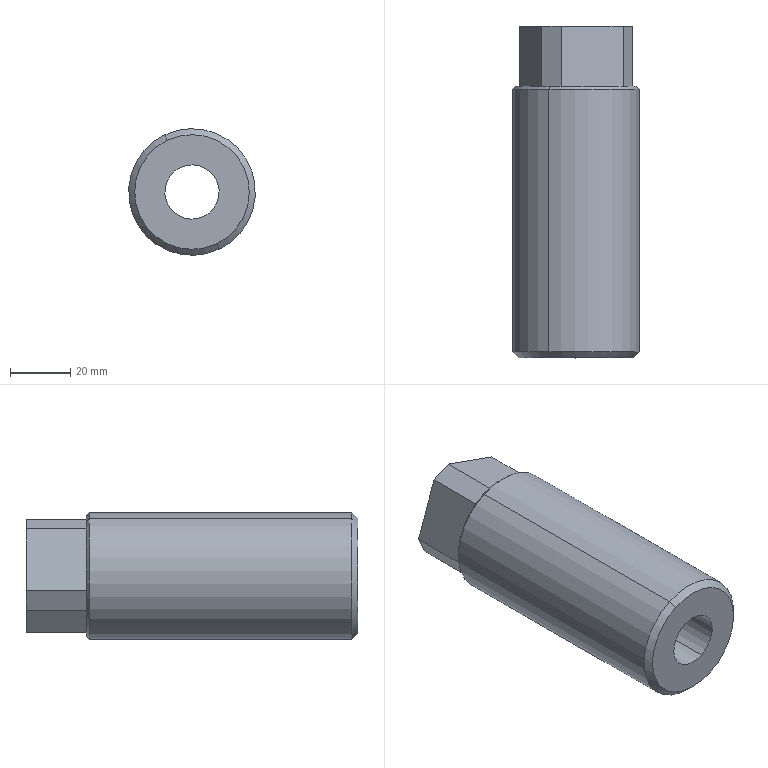Component | SolidWorks | YC1-250-02-28MotorSeatAssembly-1_YC1-200-02-29AdjustmentScrew-1 | 1 solid | 19 faces | box 42 x 110 x 42 mm | volume 115805 mm3 | plane 11 | cylinder 4 | cone 4 | commonest cylinder face diameters 42 x2 18 x2 | material Plain Carbon Steel
STEP:
#1=CARTESIAN_POINT('',(15.592,146.811,-50.827));
#2=VERTEX_POINT('',#1);
#3=CARTESIAN_POINT('',(16.298,146.811,-52.322));
#4=VERTEX_POINT('',#3);
#5=CARTESIAN_POINT('',(15.945,146.811,-51.575));
#6=DIRECTION('',(0.,-1.,0.));
#7=DIRECTION('',(-0.4273,0.,0.9041));
#8=AXIS2_PLACEMENT_3D('',#5,#6,#7);
#9=CIRCLE('',#8,0.8268);
#10=EDGE_CURVE('',#2,#4,#9,.T.);
#11=ORIENTED_EDGE('',*,*,#10,.T.);
#12=CARTESIAN_POINT('',(16.298,143.386,-52.322));
#13=VERTEX_POINT('',#12);
#14=CARTESIAN_POINT('',(16.298,147.638,-52.322));
#15=DIRECTION('',(0.,-1.,0.));
#16=VECTOR('',#15,39.37);
#17=LINE('',#14,#16);
#18=EDGE_CURVE('',#4,#13,#17,.T.);
#19=ORIENTED_EDGE('',*,*,#18,.T.);
#20=CARTESIAN_POINT('',(15.592,143.386,-50.827));
#21=VERTEX_POINT('',#20);
#22=CARTESIAN_POINT('',(15.945,143.386,-51.575));
#23=DIRECTION('',(0.,1.,0.));
#24=DIRECTION('',(-0.4273,0.,0.9041));
#25=AXIS2_PLACEMENT_3D('',#22,#23,#24);
#26=CIRCLE('',#25,0.8268);
#27=EDGE_CURVE('',#13,#21,#26,.T.);
#28=ORIENTED_EDGE('',*,*,#27,.T.);
#29=CARTESIAN_POINT('',(15.592,147.638,-50.827));
#30=DIRECTION('',(0.,-1.,0.));
#31=VECTOR('',#30,39.37);
#32=LINE('',#29,#31);
#33=EDGE_CURVE('',#2,#21,#32,.T.);
#34=ORIENTED_EDGE('',*,*,#33,.F.);
#35=EDGE_LOOP('',(#11,#19,#28,#34));
#36=FACE_OUTER_BOUND('',#35,.T.);
#37=CARTESIAN_POINT('',(15.945,147.638,-51.575));
#38=DIRECTION('',(0.,-1.,0.));
#39=DIRECTION('',(-0.4273,0.,0.9041));
#40=AXIS2_PLACEMENT_3D('',#37,#38,#39);
#41=CYLINDRICAL_SURFACE('',#40,0.8268);
#42=ADVANCED_FACE('',(#36),#41,.T.);
#43=CARTESIAN_POINT('',(16.264,143.307,-52.251));
#44=VERTEX_POINT('',#43);
#45=CARTESIAN_POINT('',(15.625,143.307,-50.898));
#46=VERTEX_POINT('',#45);
#47=CARTESIAN_POINT('',(15.945,143.307,-51.575));
#48=DIRECTION('',(0.,1.,0.));
#49=DIRECTION('',(0.4273,0.,-0.9041));
#50=AXIS2_PLACEMENT_3D('',#47,#48,#49);
#51=CIRCLE('',#50,0.748);
#52=EDGE_CURVE('',#44,#46,#51,.T.);
#53=ORIENTED_EDGE('',*,*,#52,.T.);
#54=CARTESIAN_POINT('',(15.592,143.386,-50.827));
#55=DIRECTION('',(-0.3021,0.7071,0.6393));
#56=VECTOR('',#55,39.37);
#57=LINE('',#54,#56);
#58=EDGE_CURVE('',#46,#21,#57,.T.);
#59=ORIENTED_EDGE('',*,*,#58,.T.);
#60=ORIENTED_EDGE('',*,*,#27,.F.);
#61=CARTESIAN_POINT('',(16.298,143.386,-52.322));
#62=DIRECTION('',(0.3021,0.7071,-0.6393));
#63=VECTOR('',#62,39.37);
#64=LINE('',#61,#63);
#65=EDGE_CURVE('',#44,#13,#64,.T.);
#66=ORIENTED_EDGE('',*,*,#65,.F.);
#67=EDGE_LOOP('',(#53,#59,#60,#66));
#68=FACE_OUTER_BOUND('',#67,.T.);
#69=CARTESIAN_POINT('',(15.945,143.386,-51.575));
#70=DIRECTION('',(0.,1.,0.));
#71=DIRECTION('',(0.4273,0.,-0.9041));
#72=AXIS2_PLACEMENT_3D('',#69,#70,#71);
#73=CONICAL_SURFACE('',#72,0.8268,0.7854);
#74=ADVANCED_FACE('',(#68),#73,.T.);
#75=CARTESIAN_POINT('',(15.608,146.85,-50.863));
#76=VERTEX_POINT('',#75);
#77=CARTESIAN_POINT('',(16.281,146.85,-52.287));
#78=VERTEX_POINT('',#77);
#79=CARTESIAN_POINT('',(15.945,146.85,-51.575));
#80=DIRECTION('',(0.,-1.,0.));
#81=DIRECTION('',(-0.4273,0.,0.9041));
#82=AXIS2_PLACEMENT_3D('',#79,#80,#81);
#83=CIRCLE('',#82,0.7874);
#84=EDGE_CURVE('',#76,#78,#83,.T.);
#85=ORIENTED_EDGE('',*,*,#84,.T.);
#86=CARTESIAN_POINT('',(16.298,146.811,-52.322));
#87=DIRECTION('',(0.3021,-0.7071,-0.6393));
#88=VECTOR('',#87,39.37);
#89=LINE('',#86,#88);
#90=EDGE_CURVE('',#78,#4,#89,.T.);
#91=ORIENTED_EDGE('',*,*,#90,.T.);
#92=ORIENTED_EDGE('',*,*,#10,.F.);
#93=CARTESIAN_POINT('',(15.592,146.811,-50.827));
#94=DIRECTION('',(-0.3021,-0.7071,0.6393));
#95=VECTOR('',#94,39.37);
#96=LINE('',#93,#95);
#97=EDGE_CURVE('',#76,#2,#96,.T.);
#98=ORIENTED_EDGE('',*,*,#97,.F.);
#99=EDGE_LOOP('',(#85,#91,#92,#98));
#100=FACE_OUTER_BOUND('',#99,.T.);
#101=CARTESIAN_POINT('',(15.945,146.811,-51.575));
#102=DIRECTION('',(0.,-1.,0.));
#103=DIRECTION('',(-0.4273,0.,0.9041));
#104=AXIS2_PLACEMENT_3D('',#101,#102,#103);
#105=CONICAL_SURFACE('',#104,0.8268,0.7854);
#106=ADVANCED_FACE('',(#100),#105,.T.);
#107=CARTESIAN_POINT('',(16.096,143.307,-51.895));
#108=VERTEX_POINT('',#107);
#109=CARTESIAN_POINT('',(15.793,143.307,-51.254));
#110=VERTEX_POINT('',#109);
#111=CARTESIAN_POINT('',(15.945,143.307,-51.575));
#112=DIRECTION('',(0.,-1.,0.));
#113=DIRECTION('',(0.4273,0.,-0.9041));
#114=AXIS2_PLACEMENT_3D('',#111,#112,#113);
#115=CIRCLE('',#114,0.3543);
#116=EDGE_CURVE('',#108,#110,#115,.T.);
#117=ORIENTED_EDGE('',*,*,#116,.T.);
#118=CARTESIAN_POINT('',(15.793,147.638,-51.254));
#119=VERTEX_POINT('',#118);
#120=CARTESIAN_POINT('',(15.793,147.638,-51.254));
#121=DIRECTION('',(0.,1.,0.));
#122=VECTOR('',#121,39.37);
#123=LINE('',#120,#122);
#124=EDGE_CURVE('',#110,#119,#123,.T.);
#125=ORIENTED_EDGE('',*,*,#124,.T.);
#126=CARTESIAN_POINT('',(16.096,147.638,-51.895));
#127=VERTEX_POINT('',#126);
#128=CARTESIAN_POINT('',(15.945,147.638,-51.575));
#129=DIRECTION('',(0.,-1.,0.));
#130=DIRECTION('',(0.4273,0.,-0.9041));
#131=AXIS2_PLACEMENT_3D('',#128,#129,#130);
#132=CIRCLE('',#131,0.3543);
#133=EDGE_CURVE('',#127,#119,#132,.T.);
#134=ORIENTED_EDGE('',*,*,#133,.F.);
#135=CARTESIAN_POINT('',(16.096,147.638,-51.895));
#136=DIRECTION('',(0.,1.,0.));
#137=VECTOR('',#136,39.37);
#138=LINE('',#135,#137);
#139=EDGE_CURVE('',#108,#127,#138,.T.);
#140=ORIENTED_EDGE('',*,*,#139,.F.);
#141=EDGE_LOOP('',(#117,#125,#134,#140));
#142=FACE_OUTER_BOUND('',#141,.T.);
#143=CARTESIAN_POINT('',(15.945,147.638,-51.575));
#144=DIRECTION('',(0.,1.,0.));
#145=DIRECTION('',(0.4273,0.,-0.9041));
#146=AXIS2_PLACEMENT_3D('',#143,#144,#145);
#147=CYLINDRICAL_SURFACE('',#146,0.3543);
#148=ADVANCED_FACE('',(#142),#147,.F.);
#149=ORIENTED_EDGE('',*,*,#18,.F.);
#150=CARTESIAN_POINT('',(15.945,146.811,-51.575));
#151=DIRECTION('',(0.,-1.,0.));
#152=DIRECTION('',(-0.4273,0.,0.9041));
#153=AXIS2_PLACEMENT_3D('',#150,#151,#152);
#154=CIRCLE('',#153,0.8268);
#155=EDGE_CURVE('',#4,#2,#154,.T.);
#156=ORIENTED_EDGE('',*,*,#155,.T.);
#157=ORIENTED_EDGE('',*,*,#33,.T.);
#158=CARTESIAN_POINT('',(15.945,143.386,-51.575));
#159=DIRECTION('',(0.,1.,0.));
#160=DIRECTION('',(-0.4273,0.,0.9041));
#161=AXIS2_PLACEMENT_3D('',#158,#159,#160);
#162=CIRCLE('',#161,0.8268);
#163=EDGE_CURVE('',#21,#13,#162,.T.);
#164=ORIENTED_EDGE('',*,*,#163,.T.);
#165=EDGE_LOOP('',(#149,#156,#157,#164));
#166=FACE_OUTER_BOUND('',#165,.T.);
#167=CARTESIAN_POINT('',(15.945,147.638,-51.575));
#168=DIRECTION('',(0.,-1.,0.));
#169=DIRECTION('',(-0.4273,0.,0.9041));
#170=AXIS2_PLACEMENT_3D('',#167,#168,#169);
#171=CYLINDRICAL_SURFACE('',#170,0.8268);
#172=ADVANCED_FACE('',(#166),#171,.T.);
#173=ORIENTED_EDGE('',*,*,#58,.F.);
#174=CARTESIAN_POINT('',(15.945,143.307,-51.575));
#175=DIRECTION('',(0.,1.,0.));
#176=DIRECTION('',(0.4273,0.,-0.9041));
#177=AXIS2_PLACEMENT_3D('',#174,#175,#176);
#178=CIRCLE('',#177,0.748);
#179=EDGE_CURVE('',#46,#44,#178,.T.);
#180=ORIENTED_EDGE('',*,*,#179,.T.);
#181=ORIENTED_EDGE('',*,*,#65,.T.);
#182=ORIENTED_EDGE('',*,*,#163,.F.);
#183=EDGE_LOOP('',(#173,#180,#181,#182));
#184=FACE_OUTER_BOUND('',#183,.T.);
#185=CARTESIAN_POINT('',(15.945,143.386,-51.575));
#186=DIRECTION('',(0.,1.,0.));
#187=DIRECTION('',(0.4273,0.,-0.9041));
#188=AXIS2_PLACEMENT_3D('',#185,#186,#187);
#189=CONICAL_SURFACE('',#188,0.8268,0.7854);
#190=ADVANCED_FACE('',(#184),#189,.T.);
#191=ORIENTED_EDGE('',*,*,#90,.F.);
#192=CARTESIAN_POINT('',(15.945,146.85,-51.575));
#193=DIRECTION('',(0.,-1.,0.));
#194=DIRECTION('',(-0.4273,0.,0.9041));
#195=AXIS2_PLACEMENT_3D('',#192,#193,#194);
#196=CIRCLE('',#195,0.7874);
#197=EDGE_CURVE('',#78,#76,#196,.T.);
#198=ORIENTED_EDGE('',*,*,#197,.T.);
#199=ORIENTED_EDGE('',*,*,#97,.T.);
#200=ORIENTED_EDGE('',*,*,#155,.F.);
#201=EDGE_LOOP('',(#191,#198,#199,#200));
#202=FACE_OUTER_BOUND('',#201,.T.);
#203=CARTESIAN_POINT('',(15.945,146.811,-51.575));
#204=DIRECTION('',(0.,-1.,0.));
#205=DIRECTION('',(-0.4273,0.,0.9041));
#206=AXIS2_PLACEMENT_3D('',#203,#204,#205);
#207=CONICAL_SURFACE('',#206,0.8268,0.7854);
#208=ADVANCED_FACE('',(#202),#207,.T.);
#209=ORIENTED_EDGE('',*,*,#116,.F.);
#210=CARTESIAN_POINT('',(15.945,143.307,-51.575));
#211=DIRECTION('',(0.,-1.,0.));
#212=DIRECTION('',(0.4273,0.,-0.9041));
#213=AXIS2_PLACEMENT_3D('',#210,#211,#212);
#214=CIRCLE('',#213,0.3543);
#215=EDGE_CURVE('',#110,#108,#214,.T.);
#216=ORIENTED_EDGE('',*,*,#215,.F.);
#217=EDGE_LOOP('',(#209,#216));
#218=FACE_BOUND('',#217,.T.);
#219=ORIENTED_EDGE('',*,*,#52,.F.);
#220=ORIENTED_EDGE('',*,*,#179,.F.);
#221=EDGE_LOOP('',(#219,#220));
#222=FACE_OUTER_BOUND('',#221,.T.);
#223=CARTESIAN_POINT('',(15.945,143.307,-51.575));
#224=DIRECTION('',(0.,1.,0.));
#225=DIRECTION('',(0.4273,0.,-0.9041));
#226=AXIS2_PLACEMENT_3D('',#223,#224,#225);
#227=PLANE('',#226);
#228=ADVANCED_FACE('',(#218,#222),#227,.F.);
#229=CARTESIAN_POINT('',(16.682,146.85,-51.384));
#230=VERTEX_POINT('',#229);
#231=CARTESIAN_POINT('',(16.56,146.85,-51.126));
#232=VERTEX_POINT('',#231);
#233=CARTESIAN_POINT('',(16.621,146.85,-51.255));
#234=DIRECTION('',(-0.4273,0.,0.9041));
#235=VECTOR('',#234,39.37);
#236=LINE('',#233,#235);
#237=EDGE_CURVE('',#230,#232,#236,.T.);
#238=ORIENTED_EDGE('',*,*,#237,.T.);
#239=CARTESIAN_POINT('',(15.754,146.85,-50.837));
#240=VERTEX_POINT('',#239);
#241=CARTESIAN_POINT('',(16.56,146.85,-51.126));
#242=DIRECTION('',(-0.9414,0.,0.3372));
#243=VECTOR('',#242,39.37);
#244=LINE('',#241,#243);
#245=EDGE_CURVE('',#232,#240,#244,.T.);
#246=ORIENTED_EDGE('',*,*,#245,.T.);
#247=CARTESIAN_POINT('',(15.496,146.85,-50.96));
#248=VERTEX_POINT('',#247);
#249=CARTESIAN_POINT('',(15.625,146.85,-50.898));
#250=DIRECTION('',(-0.9041,0.,-0.4273));
#251=VECTOR('',#250,39.37);
#252=LINE('',#249,#251);
#253=EDGE_CURVE('',#240,#248,#252,.T.);
#254=ORIENTED_EDGE('',*,*,#253,.T.);
#255=CARTESIAN_POINT('',(15.208,146.85,-51.765));
#256=VERTEX_POINT('',#255);
#257=CARTESIAN_POINT('',(15.496,146.85,-50.96));
#258=DIRECTION('',(-0.3372,0.,-0.9414));
#259=VECTOR('',#258,39.37);
#260=LINE('',#257,#259);
#261=EDGE_CURVE('',#248,#256,#260,.T.);
#262=ORIENTED_EDGE('',*,*,#261,.T.);
#263=CARTESIAN_POINT('',(15.33,146.85,-52.024));
#264=VERTEX_POINT('',#263);
#265=CARTESIAN_POINT('',(15.269,146.85,-51.894));
#266=DIRECTION('',(0.4273,0.,-0.9041));
#267=VECTOR('',#266,39.37);
#268=LINE('',#265,#267);
#269=EDGE_CURVE('',#256,#264,#268,.T.);
#270=ORIENTED_EDGE('',*,*,#269,.T.);
#271=CARTESIAN_POINT('',(16.135,146.85,-52.312));
#272=VERTEX_POINT('',#271);
#273=CARTESIAN_POINT('',(15.33,146.85,-52.024));
#274=DIRECTION('',(0.9414,0.,-0.3372));
#275=VECTOR('',#274,39.37);
#276=LINE('',#273,#275);
#277=EDGE_CURVE('',#264,#272,#276,.T.);
#278=ORIENTED_EDGE('',*,*,#277,.T.);
#279=CARTESIAN_POINT('',(16.394,146.85,-52.19));
#280=VERTEX_POINT('',#279);
#281=CARTESIAN_POINT('',(16.264,146.85,-52.251));
#282=DIRECTION('',(0.9041,0.,0.4273));
#283=VECTOR('',#282,39.37);
#284=LINE('',#281,#283);
#285=EDGE_CURVE('',#272,#280,#284,.T.);
#286=ORIENTED_EDGE('',*,*,#285,.T.);
#287=CARTESIAN_POINT('',(16.394,146.85,-52.19));
#288=DIRECTION('',(0.3372,0.,0.9414));
#289=VECTOR('',#288,39.37);
#290=LINE('',#287,#289);
#291=EDGE_CURVE('',#280,#230,#290,.T.);
#292=ORIENTED_EDGE('',*,*,#291,.T.);
#293=EDGE_LOOP('',(#238,#246,#254,#262,#270,#278,#286,#292));
#294=FACE_BOUND('',#293,.T.);
#295=ORIENTED_EDGE('',*,*,#84,.F.);
#296=ORIENTED_EDGE('',*,*,#197,.F.);
#297=EDGE_LOOP('',(#295,#296));
#298=FACE_OUTER_BOUND('',#297,.T.);
#299=CARTESIAN_POINT('',(15.945,146.85,-51.575));
#300=DIRECTION('',(0.,1.,0.));
#301=DIRECTION('',(0.4273,0.,-0.9041));
#302=AXIS2_PLACEMENT_3D('',#299,#300,#301);
#303=PLANE('',#302);
#304=ADVANCED_FACE('',(#294,#298),#303,.T.);
#305=ORIENTED_EDGE('',*,*,#124,.F.);
#306=ORIENTED_EDGE('',*,*,#215,.T.);
#307=ORIENTED_EDGE('',*,*,#139,.T.);
#308=CARTESIAN_POINT('',(15.945,147.638,-51.575));
#309=DIRECTION('',(0.,-1.,0.));
#310=DIRECTION('',(0.4273,0.,-0.9041));
#311=AXIS2_PLACEMENT_3D('',#308,#309,#310);
#312=CIRCLE('',#311,0.3543);
#313=EDGE_CURVE('',#119,#127,#312,.T.);
#314=ORIENTED_EDGE('',*,*,#313,.F.);
#315=EDGE_LOOP('',(#305,#306,#307,#314));
#316=FACE_OUTER_BOUND('',#315,.T.);
#317=CARTESIAN_POINT('',(15.945,147.638,-51.575));
#318=DIRECTION('',(0.,1.,0.));
#319=DIRECTION('',(0.4273,0.,-0.9041));
#320=AXIS2_PLACEMENT_3D('',#317,#318,#319);
#321=CYLINDRICAL_SURFACE('',#320,0.3543);
#322=ADVANCED_FACE('',(#316),#321,.F.);
#323=ORIENTED_EDGE('',*,*,#245,.F.);
#324=CARTESIAN_POINT('',(16.56,147.638,-51.126));
#325=VERTEX_POINT('',#324);
#326=CARTESIAN_POINT('',(16.56,146.85,-51.126));
#327=DIRECTION('',(0.,1.,0.));
#328=VECTOR('',#327,39.37);
#329=LINE('',#326,#328);
#330=EDGE_CURVE('',#232,#325,#329,.T.);
#331=ORIENTED_EDGE('',*,*,#330,.T.);
#332=CARTESIAN_POINT('',(15.754,147.638,-50.837));
#333=VERTEX_POINT('',#332);
#334=CARTESIAN_POINT('',(15.754,147.638,-50.837));
#335=DIRECTION('',(-0.9414,0.,0.3372));
#336=VECTOR('',#335,39.37);
#337=LINE('',#334,#336);
#338=EDGE_CURVE('',#325,#333,#337,.T.);
#339=ORIENTED_EDGE('',*,*,#338,.T.);
#340=CARTESIAN_POINT('',(15.754,146.85,-50.837));
#341=DIRECTION('',(0.,-1.,0.));
#342=VECTOR('',#341,39.37);
#343=LINE('',#340,#342);
#344=EDGE_CURVE('',#333,#240,#343,.T.);
#345=ORIENTED_EDGE('',*,*,#344,.T.);
#346=EDGE_LOOP('',(#323,#331,#339,#345));
#347=FACE_OUTER_BOUND('',#346,.T.);
#348=CARTESIAN_POINT('',(15.754,146.85,-50.837));
#349=DIRECTION('',(0.3372,0.,0.9414));
#350=DIRECTION('',(0.9414,0.,-0.3372));
#351=AXIS2_PLACEMENT_3D('',#348,#349,#350);
#352=PLANE('',#351);
#353=ADVANCED_FACE('',(#347),#352,.T.);
#354=ORIENTED_EDGE('',*,*,#237,.F.);
#355=CARTESIAN_POINT('',(16.682,147.638,-51.384));
#356=VERTEX_POINT('',#355);
#357=CARTESIAN_POINT('',(16.682,146.85,-51.384));
#358=DIRECTION('',(0.,1.,0.));
#359=VECTOR('',#358,39.37);
#360=LINE('',#357,#359);
#361=EDGE_CURVE('',#230,#356,#360,.T.);
#362=ORIENTED_EDGE('',*,*,#361,.T.);
#363=CARTESIAN_POINT('',(16.56,147.638,-51.126));
#364=DIRECTION('',(-0.4273,0.,0.9041));
#365=VECTOR('',#364,39.37);
#366=LINE('',#363,#365);
#367=EDGE_CURVE('',#356,#325,#366,.T.);
#368=ORIENTED_EDGE('',*,*,#367,.T.);
#369=ORIENTED_EDGE('',*,*,#330,.F.);
#370=EDGE_LOOP('',(#354,#362,#368,#369));
#371=FACE_OUTER_BOUND('',#370,.T.);
#372=CARTESIAN_POINT('',(16.56,146.85,-51.126));
#373=DIRECTION('',(0.9041,0.,0.4273));
#374=DIRECTION('',(0.4273,0.,-0.9041));
#375=AXIS2_PLACEMENT_3D('',#372,#373,#374);
#376=PLANE('',#375);
#377=ADVANCED_FACE('',(#371),#376,.T.);
#378=ORIENTED_EDGE('',*,*,#291,.F.);
#379=CARTESIAN_POINT('',(16.394,147.638,-52.19));
#380=VERTEX_POINT('',#379);
#381=CARTESIAN_POINT('',(16.394,146.85,-52.19));
#382=DIRECTION('',(0.,1.,0.));
#383=VECTOR('',#382,39.37);
#384=LINE('',#381,#383);
#385=EDGE_CURVE('',#280,#380,#384,.T.);
#386=ORIENTED_EDGE('',*,*,#385,.T.);
#387=CARTESIAN_POINT('',(16.682,147.638,-51.384));
#388=DIRECTION('',(0.3372,0.,0.9414));
#389=VECTOR('',#388,39.37);
#390=LINE('',#387,#389);
#391=EDGE_CURVE('',#380,#356,#390,.T.);
#392=ORIENTED_EDGE('',*,*,#391,.T.);
#393=ORIENTED_EDGE('',*,*,#361,.F.);
#394=EDGE_LOOP('',(#378,#386,#392,#393));
#395=FACE_OUTER_BOUND('',#394,.T.);
#396=CARTESIAN_POINT('',(16.682,146.85,-51.384));
#397=DIRECTION('',(0.9414,0.,-0.3372));
#398=DIRECTION('',(-0.3372,0.,-0.9414));
#399=AXIS2_PLACEMENT_3D('',#396,#397,#398);
#400=PLANE('',#399);
#401=ADVANCED_FACE('',(#395),#400,.T.);
#402=ORIENTED_EDGE('',*,*,#285,.F.);
#403=CARTESIAN_POINT('',(16.135,147.638,-52.312));
#404=VERTEX_POINT('',#403);
#405=CARTESIAN_POINT('',(16.135,146.85,-52.312));
#406=DIRECTION('',(0.,1.,0.));
#407=VECTOR('',#406,39.37);
#408=LINE('',#405,#407);
#409=EDGE_CURVE('',#272,#404,#408,.T.);
#410=ORIENTED_EDGE('',*,*,#409,.T.);
#411=CARTESIAN_POINT('',(16.394,147.638,-52.19));
#412=DIRECTION('',(0.9041,0.,0.4273));
#413=VECTOR('',#412,39.37);
#414=LINE('',#411,#413);
#415=EDGE_CURVE('',#404,#380,#414,.T.);
#416=ORIENTED_EDGE('',*,*,#415,.T.);
#417=ORIENTED_EDGE('',*,*,#385,.F.);
#418=EDGE_LOOP('',(#402,#410,#416,#417));
#419=FACE_OUTER_BOUND('',#418,.T.);
#420=CARTESIAN_POINT('',(16.394,146.85,-52.19));
#421=DIRECTION('',(0.4273,0.,-0.9041));
#422=DIRECTION('',(-0.9041,0.,-0.4273));
#423=AXIS2_PLACEMENT_3D('',#420,#421,#422);
#424=PLANE('',#423);
#425=ADVANCED_FACE('',(#419),#424,.T.);
#426=ORIENTED_EDGE('',*,*,#277,.F.);
#427=CARTESIAN_POINT('',(15.33,147.638,-52.024));
#428=VERTEX_POINT('',#427);
#429=CARTESIAN_POINT('',(15.33,146.85,-52.024));
#430=DIRECTION('',(0.,1.,0.));
#431=VECTOR('',#430,39.37);
#432=LINE('',#429,#431);
#433=EDGE_CURVE('',#264,#428,#432,.T.);
#434=ORIENTED_EDGE('',*,*,#433,.T.);
#435=CARTESIAN_POINT('',(16.135,147.638,-52.312));
#436=DIRECTION('',(0.9414,0.,-0.3372));
#437=VECTOR('',#436,39.37);
#438=LINE('',#435,#437);
#439=EDGE_CURVE('',#428,#404,#438,.T.);
#440=ORIENTED_EDGE('',*,*,#439,.T.);
#441=ORIENTED_EDGE('',*,*,#409,.F.);
#442=EDGE_LOOP('',(#426,#434,#440,#441));
#443=FACE_OUTER_BOUND('',#442,.T.);
#444=CARTESIAN_POINT('',(16.135,146.85,-52.312));
#445=DIRECTION('',(-0.3372,0.,-0.9414));
#446=DIRECTION('',(-0.9414,0.,0.3372));
#447=AXIS2_PLACEMENT_3D('',#444,#445,#446);
#448=PLANE('',#447);
#449=ADVANCED_FACE('',(#443),#448,.T.);
#450=ORIENTED_EDGE('',*,*,#269,.F.);
#451=CARTESIAN_POINT('',(15.208,147.638,-51.765));
#452=VERTEX_POINT('',#451);
#453=CARTESIAN_POINT('',(15.208,146.85,-51.765));
#454=DIRECTION('',(0.,1.,0.));
#455=VECTOR('',#454,39.37);
#456=LINE('',#453,#455);
#457=EDGE_CURVE('',#256,#452,#456,.T.);
#458=ORIENTED_EDGE('',*,*,#457,.T.);
#459=CARTESIAN_POINT('',(15.208,147.638,-51.765));
#460=DIRECTION('',(0.4273,0.,-0.9041));
#461=VECTOR('',#460,39.37);
#462=LINE('',#459,#461);
#463=EDGE_CURVE('',#452,#428,#462,.T.);
#464=ORIENTED_EDGE('',*,*,#463,.T.);
#465=ORIENTED_EDGE('',*,*,#433,.F.);
#466=EDGE_LOOP('',(#450,#458,#464,#465));
#467=FACE_OUTER_BOUND('',#466,.T.);
#468=CARTESIAN_POINT('',(15.208,146.85,-51.765));
#469=DIRECTION('',(-0.9041,0.,-0.4273));
#470=DIRECTION('',(-0.4273,0.,0.9041));
#471=AXIS2_PLACEMENT_3D('',#468,#469,#470);
#472=PLANE('',#471);
#473=ADVANCED_FACE('',(#467),#472,.T.);
#474=ORIENTED_EDGE('',*,*,#261,.F.);
#475=CARTESIAN_POINT('',(15.496,147.638,-50.96));
#476=VERTEX_POINT('',#475);
#477=CARTESIAN_POINT('',(15.496,146.85,-50.96));
#478=DIRECTION('',(0.,1.,0.));
#479=VECTOR('',#478,39.37);
#480=LINE('',#477,#479);
#481=EDGE_CURVE('',#248,#476,#480,.T.);
#482=ORIENTED_EDGE('',*,*,#481,.T.);
#483=CARTESIAN_POINT('',(15.208,147.638,-51.765));
#484=DIRECTION('',(-0.3372,0.,-0.9414));
#485=VECTOR('',#484,39.37);
#486=LINE('',#483,#485);
#487=EDGE_CURVE('',#476,#452,#486,.T.);
#488=ORIENTED_EDGE('',*,*,#487,.T.);
#489=ORIENTED_EDGE('',*,*,#457,.F.);
#490=EDGE_LOOP('',(#474,#482,#488,#489));
#491=FACE_OUTER_BOUND('',#490,.T.);
#492=CARTESIAN_POINT('',(15.208,146.85,-51.765));
#493=DIRECTION('',(-0.9414,0.,0.3372));
#494=DIRECTION('',(0.3372,0.,0.9414));
#495=AXIS2_PLACEMENT_3D('',#492,#493,#494);
#496=PLANE('',#495);
#497=ADVANCED_FACE('',(#491),#496,.T.);
#498=ORIENTED_EDGE('',*,*,#253,.F.);
#499=ORIENTED_EDGE('',*,*,#344,.F.);
#500=CARTESIAN_POINT('',(15.754,147.638,-50.837));
#501=DIRECTION('',(-0.9041,0.,-0.4273));
#502=VECTOR('',#501,39.37);
#503=LINE('',#500,#502);
#504=EDGE_CURVE('',#333,#476,#503,.T.);
#505=ORIENTED_EDGE('',*,*,#504,.T.);
#506=ORIENTED_EDGE('',*,*,#481,.F.);
#507=EDGE_LOOP('',(#498,#499,#505,#506));
#508=FACE_OUTER_BOUND('',#507,.T.);
#509=CARTESIAN_POINT('',(15.754,146.85,-50.837));
#510=DIRECTION('',(-0.4273,0.,0.9041));
#511=DIRECTION('',(0.9041,0.,0.4273));
#512=AXIS2_PLACEMENT_3D('',#509,#510,#511);
#513=PLANE('',#512);
#514=ADVANCED_FACE('',(#508),#513,.T.);
#515=ORIENTED_EDGE('',*,*,#463,.F.);
#516=ORIENTED_EDGE('',*,*,#487,.F.);
#517=ORIENTED_EDGE('',*,*,#504,.F.);
#518=ORIENTED_EDGE('',*,*,#338,.F.);
#519=ORIENTED_EDGE('',*,*,#367,.F.);
#520=ORIENTED_EDGE('',*,*,#391,.F.);
#521=ORIENTED_EDGE('',*,*,#415,.F.);
#522=ORIENTED_EDGE('',*,*,#439,.F.);
#523=EDGE_LOOP('',(#515,#516,#517,#518,#519,#520,#521,#522));
#524=FACE_OUTER_BOUND('',#523,.T.);
#525=ORIENTED_EDGE('',*,*,#133,.T.);
#526=ORIENTED_EDGE('',*,*,#313,.T.);
#527=EDGE_LOOP('',(#525,#526));
#528=FACE_BOUND('',#527,.T.);
#529=CARTESIAN_POINT('',(15.945,147.638,-51.575));
#530=DIRECTION('',(0.,1.,0.));
#531=DIRECTION('',(0.4273,0.,-0.9041));
#532=AXIS2_PLACEMENT_3D('',#529,#530,#531);
#533=PLANE('',#532);
#534=ADVANCED_FACE('',(#524,#528),#533,.T.);
#535=CLOSED_SHELL('',(#42,#74,#106,#148,#172,#190,#208,#228,#304,#322,#353,#377,#401,#425,#449,#473,#497,#514,#534));
#536=MANIFOLD_SOLID_BREP('',#535);
#537=CARTESIAN_POINT('',(0.,0.,0.));
#538=DIRECTION('',(0.,0.,1.));
#539=DIRECTION('',(1.,0.,0.));
#540=AXIS2_PLACEMENT_3D('',#537,#538,#539);
#541=(LENGTH_UNIT()NAMED_UNIT(*)SI_UNIT($,.METRE.));
#542=LENGTH_MEASURE_WITH_UNIT(LENGTH_MEASURE(0.0254),#541);
#543=DIMENSIONAL_EXPONENTS(1.,0.,0.,0.,0.,0.,0.);
#544=(CONVERSION_BASED_UNIT('',#542)LENGTH_UNIT()NAMED_UNIT(#543));
#545=UNCERTAINTY_MEASURE_WITH_UNIT(LENGTH_MEASURE(0.00001),#544,'','');
#546=(NAMED_UNIT(*)PLANE_ANGLE_UNIT()SI_UNIT($,.RADIAN.));
#547=(NAMED_UNIT(*)SI_UNIT($,.STERADIAN.)SOLID_ANGLE_UNIT());
#548=(GEOMETRIC_REPRESENTATION_CONTEXT(3)GLOBAL_UNCERTAINTY_ASSIGNED_CONTEXT((#545))GLOBAL_UNIT_ASSIGNED_CONTEXT((#544,#546,#547))REPRESENTATION_CONTEXT('',''));
#549=ADVANCED_BREP_SHAPE_REPRESENTATION('',(#536,#540),#548);
#550=COLOUR_RGB('',0.7922,0.8196,0.9333);
#551=FILL_AREA_STYLE_COLOUR('',#550);
#552=FILL_AREA_STYLE('',(#551));
#553=SURFACE_STYLE_FILL_AREA(#552);
#554=SURFACE_SIDE_STYLE('',(#553));
#555=SURFACE_STYLE_USAGE(.BOTH.,#554);
#556=PRESENTATION_STYLE_ASSIGNMENT((#555));
#557=STYLED_ITEM('',(#556),#536);
#558=PRESENTATION_LAYER_ASSIGNMENT('','',(#557));
#559=(LENGTH_UNIT()NAMED_UNIT(*)SI_UNIT($,.METRE.));
#560=LENGTH_MEASURE_WITH_UNIT(LENGTH_MEASURE(0.0254),#559);
#561=DIMENSIONAL_EXPONENTS(1.,0.,0.,0.,0.,0.,0.);
#562=(CONVERSION_BASED_UNIT('',#560)LENGTH_UNIT()NAMED_UNIT(#561));
#563=UNCERTAINTY_MEASURE_WITH_UNIT(LENGTH_MEASURE(0.00001),#562,'','');
#564=(NAMED_UNIT(*)PLANE_ANGLE_UNIT()SI_UNIT($,.RADIAN.));
#565=(NAMED_UNIT(*)SI_UNIT($,.STERADIAN.)SOLID_ANGLE_UNIT());
#566=(GEOMETRIC_REPRESENTATION_CONTEXT(3)GLOBAL_UNCERTAINTY_ASSIGNED_CONTEXT((#563))GLOBAL_UNIT_ASSIGNED_CONTEXT((#562,#564,#565))REPRESENTATION_CONTEXT('',''));
#567=MECHANICAL_DESIGN_GEOMETRIC_PRESENTATION_REPRESENTATION('',(#557),#566);